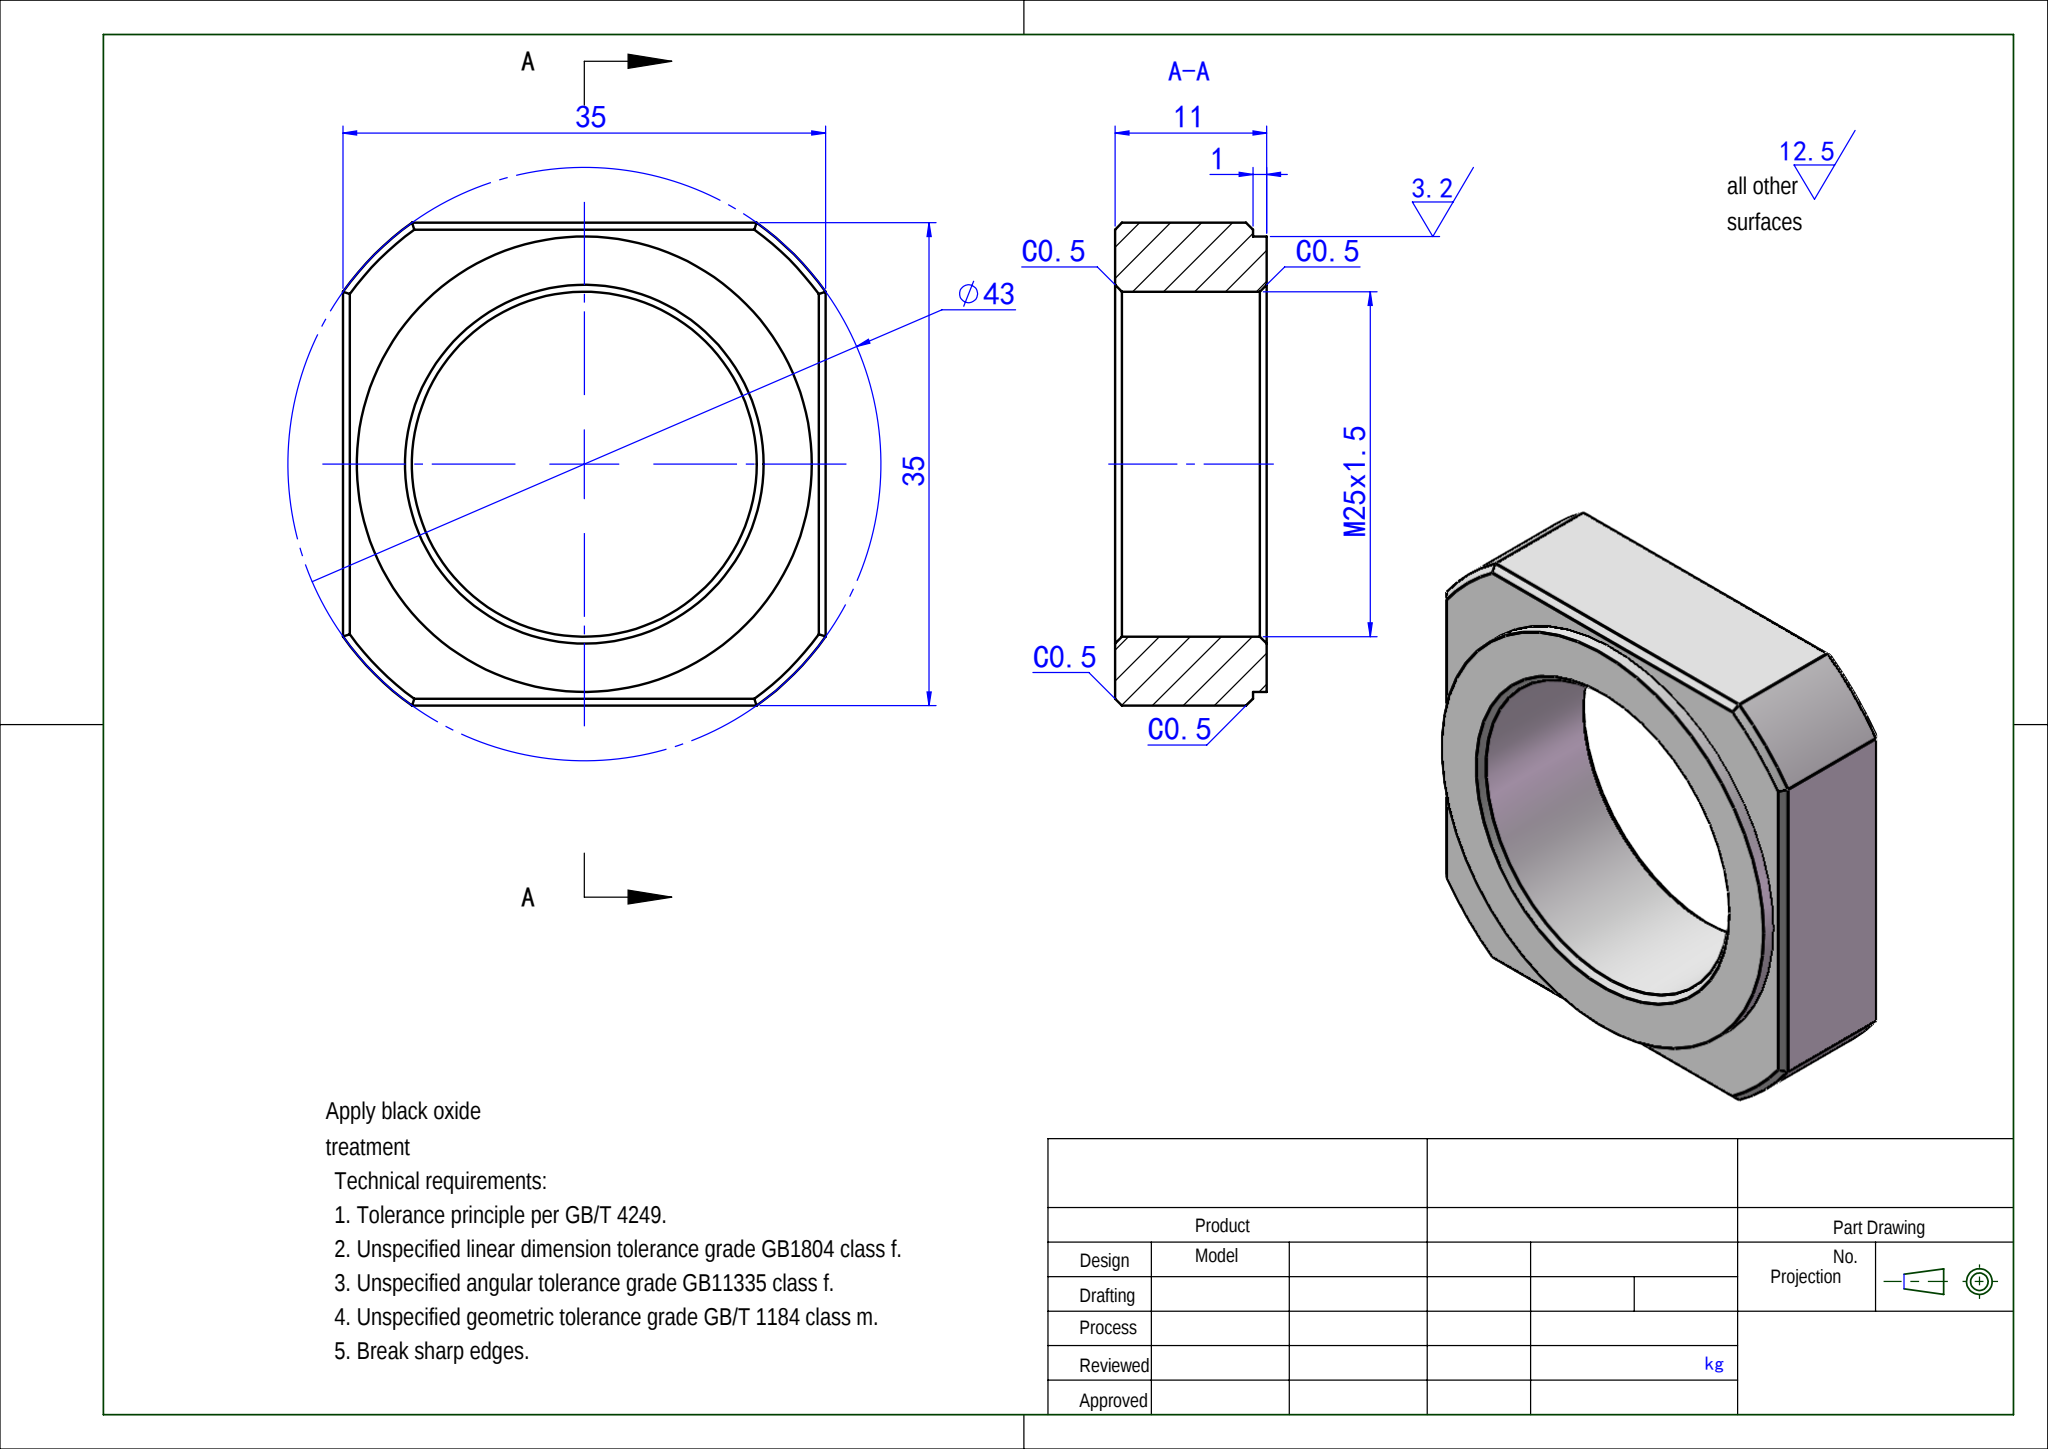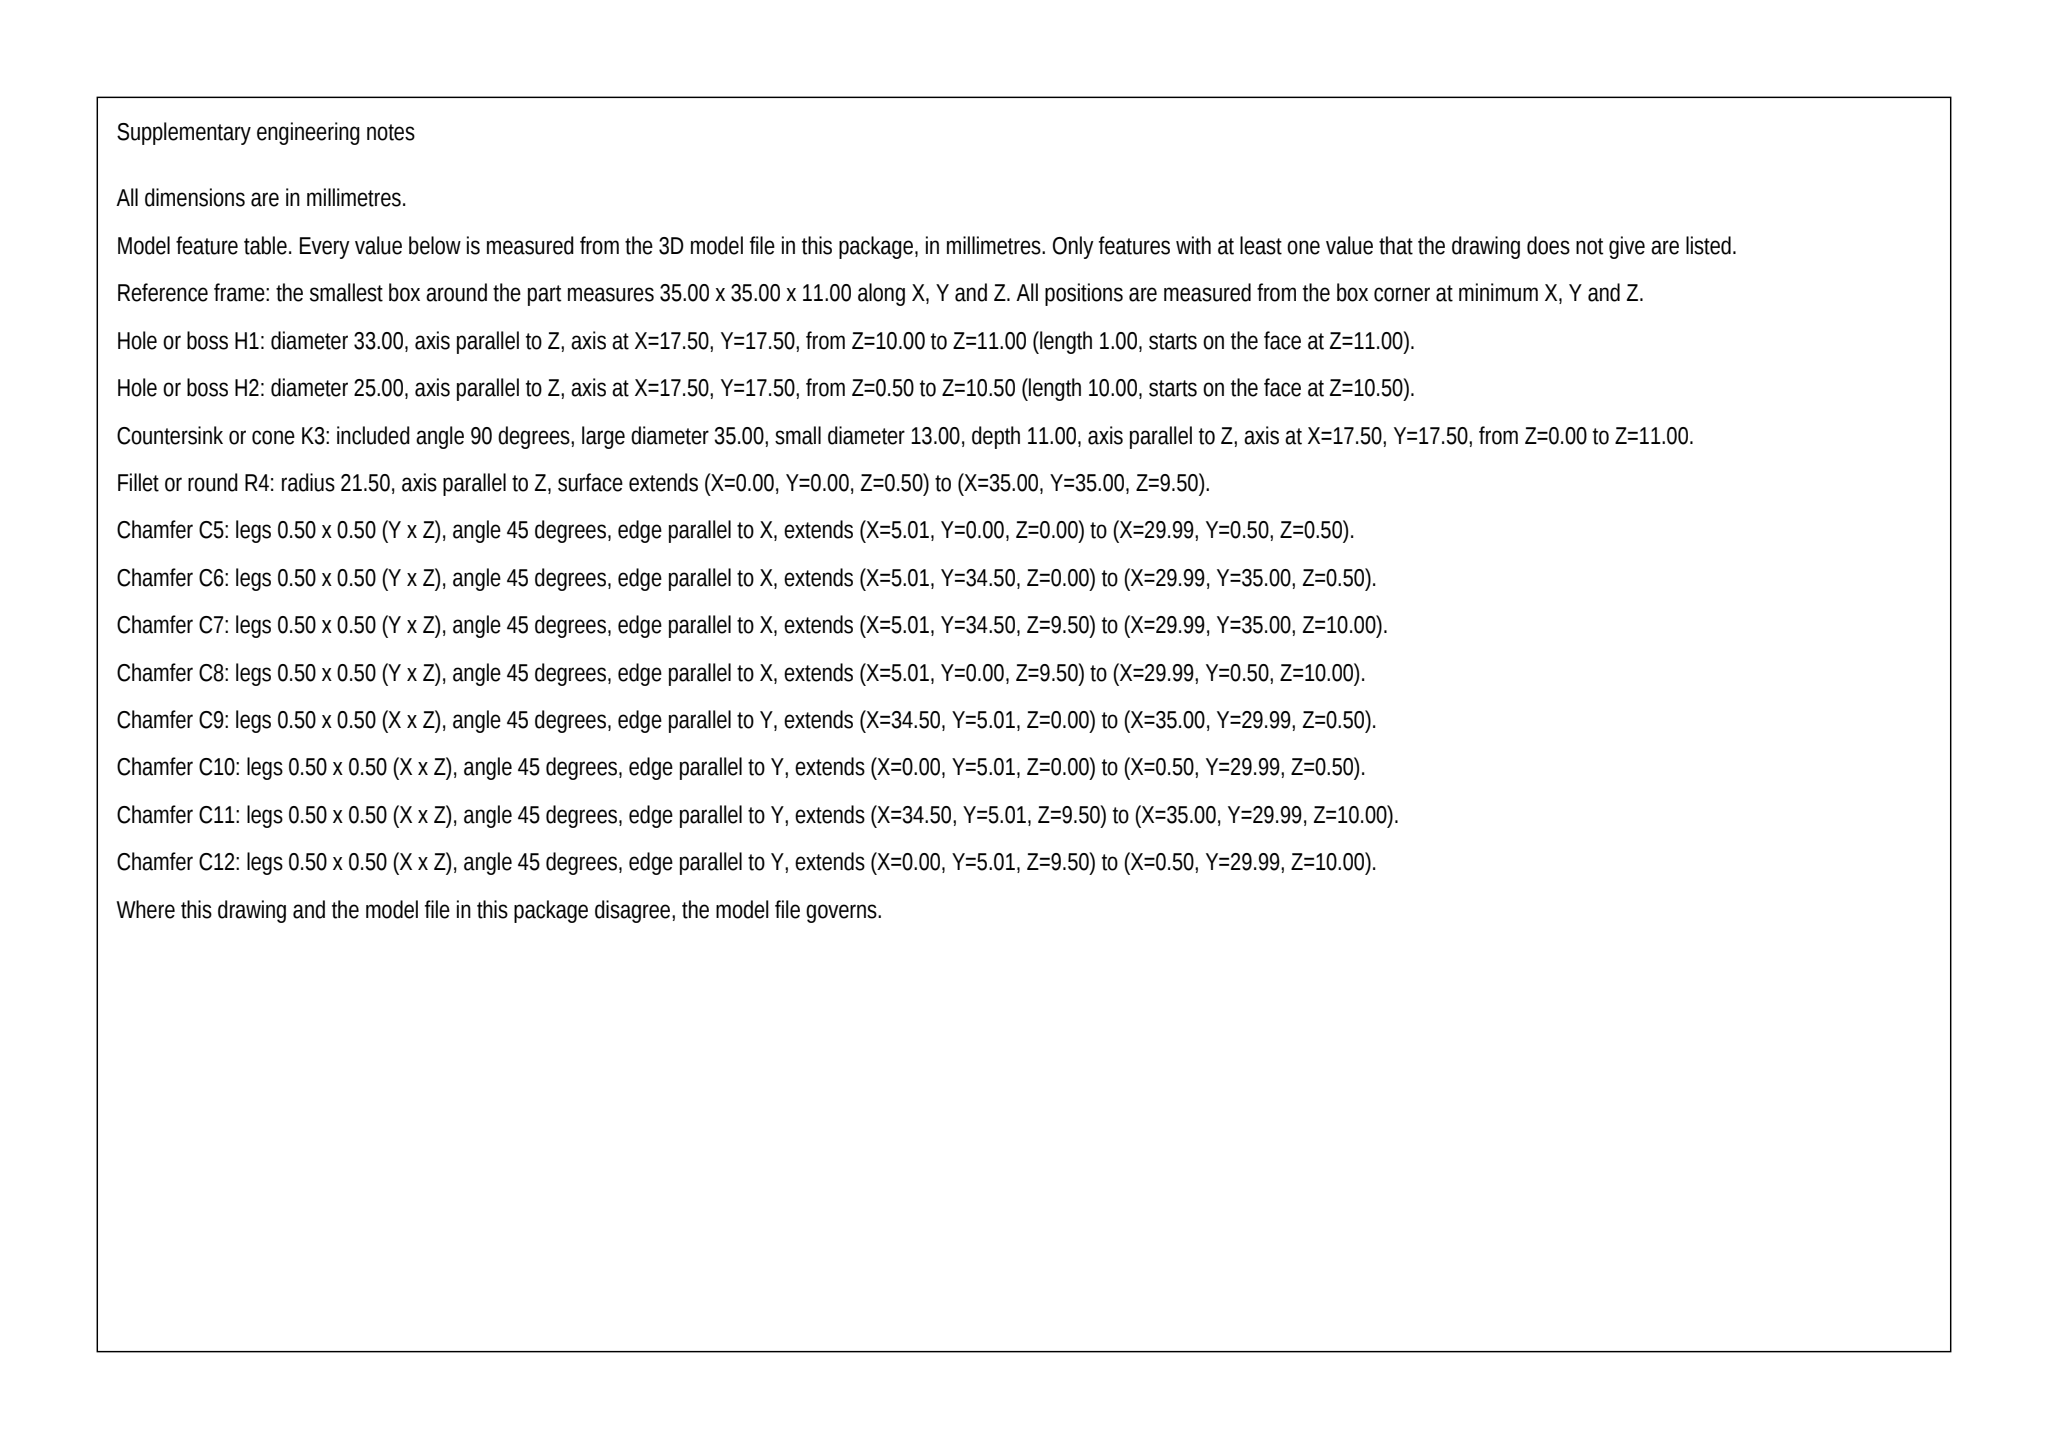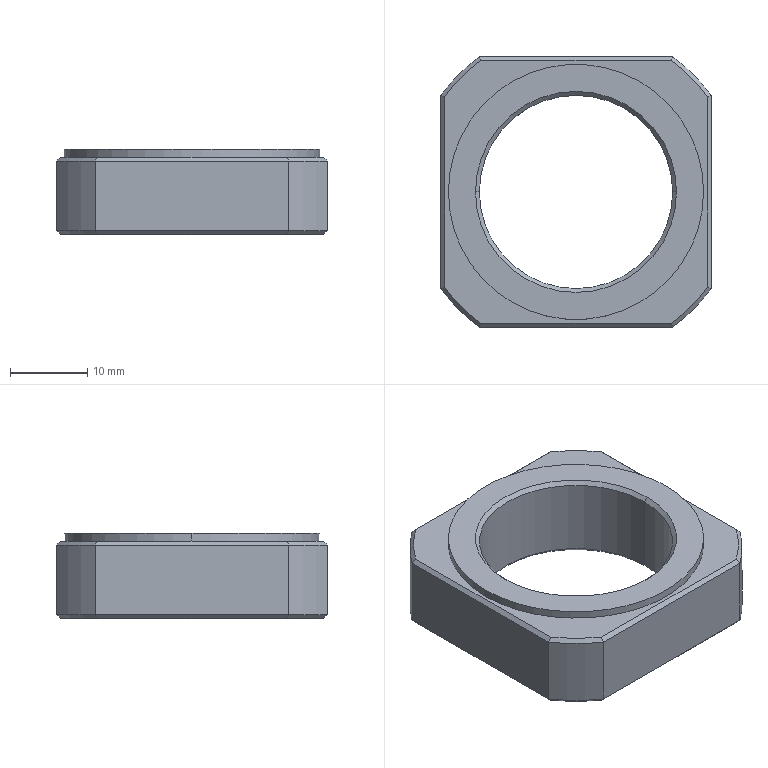Part | SolidWorks | mm | 1 solid | 35 faces | box 35 x 35 x 11 mm | volume 7208 mm3 | plane 15 | cone 12 | cylinder 8 | commonest cylinder face diameters 43 x4 33 x2 25 x2
Drawing notes:
C'BORE Ø33 DP 1 THIS END (BOTH ENDS), CONC W/ M25x1.5 | from the solid: cyl dia 33, axis z at (17.5,17.5), length 1.0, count 2; z planes at 10.0 and 11.0 with total thk 11 => 1 deep recess each end